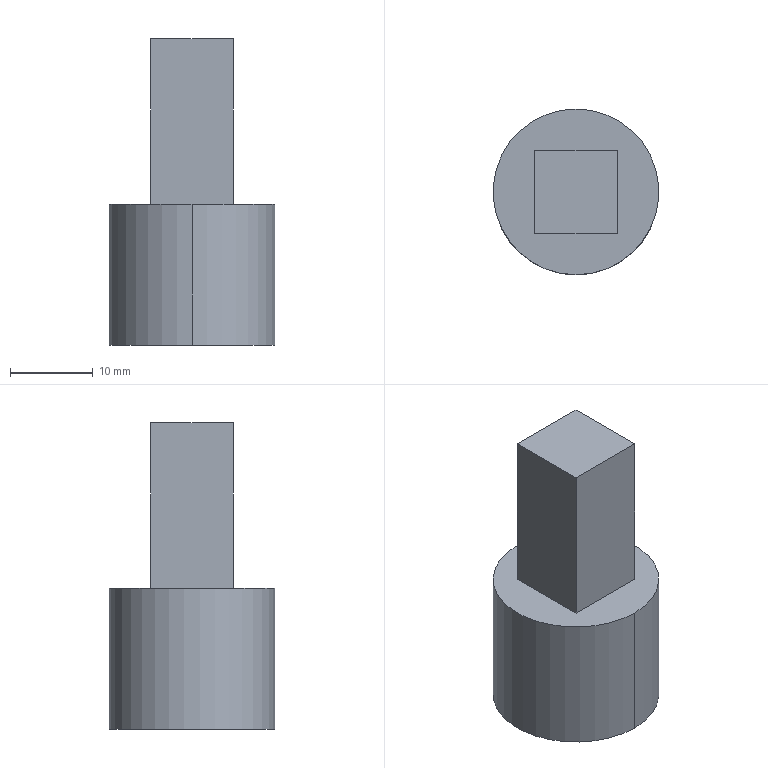Component | SolidWorks | MotorDriveShaft-1 | 1 solid | 12 faces | box 20 x 20 x 37 mm | volume 5032 mm3 | plane 8 | cylinder 4 | commonest cylinder face diameters 14 x2 20 x2
build123d program:
from build123d import *

# Parameters (mm, degrees)
SKETCH1_W           = 10
SKETCH1_H           = 10
BOSS_EXTRUDE1_DEPTH = 20
SKETCH2_R           = 10
BOSS_EXTRUDE2_DEPTH = 2
SKETCH3_R           = 10
SKETCH3_R_2         = 7
BOSS_EXTRUDE3_DEPTH = 15


with BuildPart() as part:
    # Sketch1 → Boss-Extrude1 (new body)
    with BuildSketch(Plane.XY):
        Rectangle(SKETCH1_W, SKETCH1_H)
    extrude(amount=BOSS_EXTRUDE1_DEPTH)

    # Sketch2 → Boss-Extrude2 (add)
    with BuildSketch(Plane.XY.offset(20)):
        Circle(SKETCH2_R)
    extrude(amount=BOSS_EXTRUDE2_DEPTH)

    # Sketch3 → Boss-Extrude3 (add)
    with BuildSketch(Plane.XY.offset(22)):
        Circle(SKETCH3_R)
        Circle(SKETCH3_R_2, mode=Mode.SUBTRACT)
    extrude(amount=BOSS_EXTRUDE3_DEPTH)


solid = part.part

# Placed as in the assembly
solid = solid.moved(Location((-65.193, -32.853, 1589.064), (180, 0, 0)))
STEP:
#1=CARTESIAN_POINT('',(-2.567,-1.018,61.105));
#2=VERTEX_POINT('',#1);
#3=CARTESIAN_POINT('',(-2.567,-1.569,61.105));
#4=VERTEX_POINT('',#3);
#5=CARTESIAN_POINT('',(-2.567,-1.293,61.105));
#6=DIRECTION('',(-0.,-0.,-1.));
#7=DIRECTION('',(0.,-1.,0.));
#8=AXIS2_PLACEMENT_3D('',#5,#6,#7);
#9=CIRCLE('',#8,0.2756);
#10=EDGE_CURVE('',#2,#4,#9,.T.);
#11=ORIENTED_EDGE('',*,*,#10,.T.);
#12=CARTESIAN_POINT('',(-2.567,-1.569,61.695));
#13=VERTEX_POINT('',#12);
#14=CARTESIAN_POINT('',(-2.567,-1.569,61.105));
#15=DIRECTION('',(0.,0.,1.));
#16=VECTOR('',#15,39.37);
#17=LINE('',#14,#16);
#18=EDGE_CURVE('',#4,#13,#17,.T.);
#19=ORIENTED_EDGE('',*,*,#18,.T.);
#20=CARTESIAN_POINT('',(-2.567,-1.018,61.695));
#21=VERTEX_POINT('',#20);
#22=CARTESIAN_POINT('',(-2.567,-1.293,61.695));
#23=DIRECTION('',(0.,0.,1.));
#24=DIRECTION('',(0.,-1.,0.));
#25=AXIS2_PLACEMENT_3D('',#22,#23,#24);
#26=CIRCLE('',#25,0.2756);
#27=EDGE_CURVE('',#13,#21,#26,.T.);
#28=ORIENTED_EDGE('',*,*,#27,.T.);
#29=CARTESIAN_POINT('',(-2.567,-1.018,61.105));
#30=DIRECTION('',(0.,0.,1.));
#31=VECTOR('',#30,39.37);
#32=LINE('',#29,#31);
#33=EDGE_CURVE('',#2,#21,#32,.T.);
#34=ORIENTED_EDGE('',*,*,#33,.F.);
#35=EDGE_LOOP('',(#11,#19,#28,#34));
#36=FACE_OUTER_BOUND('',#35,.T.);
#37=CARTESIAN_POINT('',(-2.567,-1.293,61.105));
#38=DIRECTION('',(0.,0.,1.));
#39=DIRECTION('',(0.,1.,0.));
#40=AXIS2_PLACEMENT_3D('',#37,#38,#39);
#41=CYLINDRICAL_SURFACE('',#40,0.2756);
#42=ADVANCED_FACE('',(#36),#41,.F.);
#43=CARTESIAN_POINT('',(-2.567,-1.687,61.105));
#44=VERTEX_POINT('',#43);
#45=CARTESIAN_POINT('',(-2.567,-0.8997,61.105));
#46=VERTEX_POINT('',#45);
#47=CARTESIAN_POINT('',(-2.567,-1.293,61.105));
#48=DIRECTION('',(-0.,-0.,-1.));
#49=DIRECTION('',(0.,-1.,0.));
#50=AXIS2_PLACEMENT_3D('',#47,#48,#49);
#51=CIRCLE('',#50,0.3937);
#52=EDGE_CURVE('',#44,#46,#51,.T.);
#53=ORIENTED_EDGE('',*,*,#52,.F.);
#54=CARTESIAN_POINT('',(-2.567,-1.687,61.774));
#55=VERTEX_POINT('',#54);
#56=CARTESIAN_POINT('',(-2.567,-1.687,61.695));
#57=DIRECTION('',(0.,0.,1.));
#58=VECTOR('',#57,39.37);
#59=LINE('',#56,#58);
#60=EDGE_CURVE('',#44,#55,#59,.T.);
#61=ORIENTED_EDGE('',*,*,#60,.T.);
#62=CARTESIAN_POINT('',(-2.567,-0.8997,61.774));
#63=VERTEX_POINT('',#62);
#64=CARTESIAN_POINT('',(-2.567,-1.293,61.774));
#65=DIRECTION('',(-0.,-0.,-1.));
#66=DIRECTION('',(0.,-1.,0.));
#67=AXIS2_PLACEMENT_3D('',#64,#65,#66);
#68=CIRCLE('',#67,0.3937);
#69=EDGE_CURVE('',#55,#63,#68,.T.);
#70=ORIENTED_EDGE('',*,*,#69,.T.);
#71=CARTESIAN_POINT('',(-2.567,-0.8997,61.695));
#72=DIRECTION('',(0.,0.,1.));
#73=VECTOR('',#72,39.37);
#74=LINE('',#71,#73);
#75=EDGE_CURVE('',#46,#63,#74,.T.);
#76=ORIENTED_EDGE('',*,*,#75,.F.);
#77=EDGE_LOOP('',(#53,#61,#70,#76));
#78=FACE_OUTER_BOUND('',#77,.T.);
#79=CARTESIAN_POINT('',(-2.567,-1.293,61.695));
#80=DIRECTION('',(0.,0.,1.));
#81=DIRECTION('',(0.,1.,0.));
#82=AXIS2_PLACEMENT_3D('',#79,#80,#81);
#83=CYLINDRICAL_SURFACE('',#82,0.3937);
#84=ADVANCED_FACE('',(#78),#83,.T.);
#85=CARTESIAN_POINT('',(-2.37,-1.49,62.562));
#86=VERTEX_POINT('',#85);
#87=CARTESIAN_POINT('',(-2.764,-1.49,62.562));
#88=VERTEX_POINT('',#87);
#89=CARTESIAN_POINT('',(-2.764,-1.49,62.562));
#90=DIRECTION('',(-1.,0.,0.));
#91=VECTOR('',#90,39.37);
#92=LINE('',#89,#91);
#93=EDGE_CURVE('',#86,#88,#92,.T.);
#94=ORIENTED_EDGE('',*,*,#93,.T.);
#95=CARTESIAN_POINT('',(-2.764,-1.49,61.774));
#96=VERTEX_POINT('',#95);
#97=CARTESIAN_POINT('',(-2.764,-1.49,61.774));
#98=DIRECTION('',(0.,0.,1.));
#99=VECTOR('',#98,39.37);
#100=LINE('',#97,#99);
#101=EDGE_CURVE('',#96,#88,#100,.T.);
#102=ORIENTED_EDGE('',*,*,#101,.F.);
#103=CARTESIAN_POINT('',(-2.37,-1.49,61.774));
#104=VERTEX_POINT('',#103);
#105=CARTESIAN_POINT('',(-2.764,-1.49,61.774));
#106=DIRECTION('',(-1.,0.,0.));
#107=VECTOR('',#106,39.37);
#108=LINE('',#105,#107);
#109=EDGE_CURVE('',#104,#96,#108,.T.);
#110=ORIENTED_EDGE('',*,*,#109,.F.);
#111=CARTESIAN_POINT('',(-2.37,-1.49,61.774));
#112=DIRECTION('',(0.,0.,1.));
#113=VECTOR('',#112,39.37);
#114=LINE('',#111,#113);
#115=EDGE_CURVE('',#104,#86,#114,.T.);
#116=ORIENTED_EDGE('',*,*,#115,.T.);
#117=EDGE_LOOP('',(#94,#102,#110,#116));
#118=FACE_OUTER_BOUND('',#117,.T.);
#119=CARTESIAN_POINT('',(-2.764,-1.49,61.774));
#120=DIRECTION('',(0.,1.,-0.));
#121=DIRECTION('',(1.,-0.,-0.));
#122=AXIS2_PLACEMENT_3D('',#119,#120,#121);
#123=PLANE('',#122);
#124=ADVANCED_FACE('',(#118),#123,.F.);
#125=CARTESIAN_POINT('',(-2.764,-1.097,62.562));
#126=VERTEX_POINT('',#125);
#127=CARTESIAN_POINT('',(-2.764,-1.097,62.562));
#128=DIRECTION('',(-0.,1.,-0.));
#129=VECTOR('',#128,39.37);
#130=LINE('',#127,#129);
#131=EDGE_CURVE('',#88,#126,#130,.T.);
#132=ORIENTED_EDGE('',*,*,#131,.T.);
#133=CARTESIAN_POINT('',(-2.764,-1.097,61.774));
#134=VERTEX_POINT('',#133);
#135=CARTESIAN_POINT('',(-2.764,-1.097,61.774));
#136=DIRECTION('',(0.,0.,1.));
#137=VECTOR('',#136,39.37);
#138=LINE('',#135,#137);
#139=EDGE_CURVE('',#134,#126,#138,.T.);
#140=ORIENTED_EDGE('',*,*,#139,.F.);
#141=CARTESIAN_POINT('',(-2.764,-1.097,61.774));
#142=DIRECTION('',(-0.,1.,-0.));
#143=VECTOR('',#142,39.37);
#144=LINE('',#141,#143);
#145=EDGE_CURVE('',#96,#134,#144,.T.);
#146=ORIENTED_EDGE('',*,*,#145,.F.);
#147=ORIENTED_EDGE('',*,*,#101,.T.);
#148=EDGE_LOOP('',(#132,#140,#146,#147));
#149=FACE_OUTER_BOUND('',#148,.T.);
#150=CARTESIAN_POINT('',(-2.764,-1.097,61.774));
#151=DIRECTION('',(1.,0.,-0.));
#152=DIRECTION('',(0.,-1.,0.));
#153=AXIS2_PLACEMENT_3D('',#150,#151,#152);
#154=PLANE('',#153);
#155=ADVANCED_FACE('',(#149),#154,.F.);
#156=CARTESIAN_POINT('',(-2.37,-1.097,62.562));
#157=VERTEX_POINT('',#156);
#158=CARTESIAN_POINT('',(-2.764,-1.097,62.562));
#159=DIRECTION('',(1.,-0.,-0.));
#160=VECTOR('',#159,39.37);
#161=LINE('',#158,#160);
#162=EDGE_CURVE('',#126,#157,#161,.T.);
#163=ORIENTED_EDGE('',*,*,#162,.T.);
#164=CARTESIAN_POINT('',(-2.37,-1.097,61.774));
#165=VERTEX_POINT('',#164);
#166=CARTESIAN_POINT('',(-2.37,-1.097,61.774));
#167=DIRECTION('',(0.,0.,1.));
#168=VECTOR('',#167,39.37);
#169=LINE('',#166,#168);
#170=EDGE_CURVE('',#165,#157,#169,.T.);
#171=ORIENTED_EDGE('',*,*,#170,.F.);
#172=CARTESIAN_POINT('',(-2.764,-1.097,61.774));
#173=DIRECTION('',(1.,-0.,-0.));
#174=VECTOR('',#173,39.37);
#175=LINE('',#172,#174);
#176=EDGE_CURVE('',#134,#165,#175,.T.);
#177=ORIENTED_EDGE('',*,*,#176,.F.);
#178=ORIENTED_EDGE('',*,*,#139,.T.);
#179=EDGE_LOOP('',(#163,#171,#177,#178));
#180=FACE_OUTER_BOUND('',#179,.T.);
#181=CARTESIAN_POINT('',(-2.764,-1.097,61.774));
#182=DIRECTION('',(-0.,-1.,0.));
#183=DIRECTION('',(-1.,0.,0.));
#184=AXIS2_PLACEMENT_3D('',#181,#182,#183);
#185=PLANE('',#184);
#186=ADVANCED_FACE('',(#180),#185,.F.);
#187=CARTESIAN_POINT('',(-2.37,-1.097,62.562));
#188=DIRECTION('',(-0.,-1.,0.));
#189=VECTOR('',#188,39.37);
#190=LINE('',#187,#189);
#191=EDGE_CURVE('',#157,#86,#190,.T.);
#192=ORIENTED_EDGE('',*,*,#191,.T.);
#193=ORIENTED_EDGE('',*,*,#115,.F.);
#194=CARTESIAN_POINT('',(-2.37,-1.097,61.774));
#195=DIRECTION('',(-0.,-1.,0.));
#196=VECTOR('',#195,39.37);
#197=LINE('',#194,#196);
#198=EDGE_CURVE('',#165,#104,#197,.T.);
#199=ORIENTED_EDGE('',*,*,#198,.F.);
#200=ORIENTED_EDGE('',*,*,#170,.T.);
#201=EDGE_LOOP('',(#192,#193,#199,#200));
#202=FACE_OUTER_BOUND('',#201,.T.);
#203=CARTESIAN_POINT('',(-2.37,-1.097,61.774));
#204=DIRECTION('',(-1.,0.,0.));
#205=DIRECTION('',(-0.,-0.,-1.));
#206=AXIS2_PLACEMENT_3D('',#203,#204,#205);
#207=PLANE('',#206);
#208=ADVANCED_FACE('',(#202),#207,.F.);
#209=ORIENTED_EDGE('',*,*,#93,.F.);
#210=ORIENTED_EDGE('',*,*,#191,.F.);
#211=ORIENTED_EDGE('',*,*,#162,.F.);
#212=ORIENTED_EDGE('',*,*,#131,.F.);
#213=EDGE_LOOP('',(#209,#210,#211,#212));
#214=FACE_OUTER_BOUND('',#213,.T.);
#215=CARTESIAN_POINT('',(-2.567,-1.293,62.562));
#216=DIRECTION('',(-0.,-0.,-1.));
#217=DIRECTION('',(-0.,-1.,0.));
#218=AXIS2_PLACEMENT_3D('',#215,#216,#217);
#219=PLANE('',#218);
#220=ADVANCED_FACE('',(#214),#219,.F.);
#221=CARTESIAN_POINT('',(-2.567,-1.293,61.774));
#222=DIRECTION('',(-0.,-0.,-1.));
#223=DIRECTION('',(0.,-1.,0.));
#224=AXIS2_PLACEMENT_3D('',#221,#222,#223);
#225=CIRCLE('',#224,0.3937);
#226=EDGE_CURVE('',#63,#55,#225,.T.);
#227=ORIENTED_EDGE('',*,*,#226,.F.);
#228=ORIENTED_EDGE('',*,*,#69,.F.);
#229=EDGE_LOOP('',(#227,#228));
#230=FACE_OUTER_BOUND('',#229,.T.);
#231=ORIENTED_EDGE('',*,*,#198,.T.);
#232=ORIENTED_EDGE('',*,*,#109,.T.);
#233=ORIENTED_EDGE('',*,*,#145,.T.);
#234=ORIENTED_EDGE('',*,*,#176,.T.);
#235=EDGE_LOOP('',(#231,#232,#233,#234));
#236=FACE_BOUND('',#235,.T.);
#237=CARTESIAN_POINT('',(-2.567,-1.293,61.774));
#238=DIRECTION('',(-0.,-0.,-1.));
#239=DIRECTION('',(-0.,-1.,0.));
#240=AXIS2_PLACEMENT_3D('',#237,#238,#239);
#241=PLANE('',#240);
#242=ADVANCED_FACE('',(#230,#236),#241,.F.);
#243=ORIENTED_EDGE('',*,*,#60,.F.);
#244=CARTESIAN_POINT('',(-2.567,-1.293,61.105));
#245=DIRECTION('',(-0.,-0.,-1.));
#246=DIRECTION('',(0.,-1.,0.));
#247=AXIS2_PLACEMENT_3D('',#244,#245,#246);
#248=CIRCLE('',#247,0.3937);
#249=EDGE_CURVE('',#46,#44,#248,.T.);
#250=ORIENTED_EDGE('',*,*,#249,.F.);
#251=ORIENTED_EDGE('',*,*,#75,.T.);
#252=ORIENTED_EDGE('',*,*,#226,.T.);
#253=EDGE_LOOP('',(#243,#250,#251,#252));
#254=FACE_OUTER_BOUND('',#253,.T.);
#255=CARTESIAN_POINT('',(-2.567,-1.293,61.695));
#256=DIRECTION('',(0.,0.,1.));
#257=DIRECTION('',(0.,1.,0.));
#258=AXIS2_PLACEMENT_3D('',#255,#256,#257);
#259=CYLINDRICAL_SURFACE('',#258,0.3937);
#260=ADVANCED_FACE('',(#254),#259,.T.);
#261=ORIENTED_EDGE('',*,*,#249,.T.);
#262=ORIENTED_EDGE('',*,*,#52,.T.);
#263=EDGE_LOOP('',(#261,#262));
#264=FACE_OUTER_BOUND('',#263,.T.);
#265=ORIENTED_EDGE('',*,*,#10,.F.);
#266=CARTESIAN_POINT('',(-2.567,-1.293,61.105));
#267=DIRECTION('',(-0.,-0.,-1.));
#268=DIRECTION('',(0.,-1.,0.));
#269=AXIS2_PLACEMENT_3D('',#266,#267,#268);
#270=CIRCLE('',#269,0.2756);
#271=EDGE_CURVE('',#4,#2,#270,.T.);
#272=ORIENTED_EDGE('',*,*,#271,.F.);
#273=EDGE_LOOP('',(#265,#272));
#274=FACE_BOUND('',#273,.T.);
#275=CARTESIAN_POINT('',(-2.567,-1.293,61.105));
#276=DIRECTION('',(-0.,-0.,-1.));
#277=DIRECTION('',(-0.,-1.,0.));
#278=AXIS2_PLACEMENT_3D('',#275,#276,#277);
#279=PLANE('',#278);
#280=ADVANCED_FACE('',(#264,#274),#279,.T.);
#281=ORIENTED_EDGE('',*,*,#18,.F.);
#282=ORIENTED_EDGE('',*,*,#271,.T.);
#283=ORIENTED_EDGE('',*,*,#33,.T.);
#284=CARTESIAN_POINT('',(-2.567,-1.293,61.695));
#285=DIRECTION('',(0.,0.,1.));
#286=DIRECTION('',(0.,-1.,0.));
#287=AXIS2_PLACEMENT_3D('',#284,#285,#286);
#288=CIRCLE('',#287,0.2756);
#289=EDGE_CURVE('',#21,#13,#288,.T.);
#290=ORIENTED_EDGE('',*,*,#289,.T.);
#291=EDGE_LOOP('',(#281,#282,#283,#290));
#292=FACE_OUTER_BOUND('',#291,.T.);
#293=CARTESIAN_POINT('',(-2.567,-1.293,61.105));
#294=DIRECTION('',(0.,0.,1.));
#295=DIRECTION('',(0.,1.,0.));
#296=AXIS2_PLACEMENT_3D('',#293,#294,#295);
#297=CYLINDRICAL_SURFACE('',#296,0.2756);
#298=ADVANCED_FACE('',(#292),#297,.F.);
#299=ORIENTED_EDGE('',*,*,#289,.F.);
#300=ORIENTED_EDGE('',*,*,#27,.F.);
#301=EDGE_LOOP('',(#299,#300));
#302=FACE_OUTER_BOUND('',#301,.T.);
#303=CARTESIAN_POINT('',(-2.567,-1.293,61.695));
#304=DIRECTION('',(-0.,-0.,-1.));
#305=DIRECTION('',(-0.,-1.,0.));
#306=AXIS2_PLACEMENT_3D('',#303,#304,#305);
#307=PLANE('',#306);
#308=ADVANCED_FACE('',(#302),#307,.T.);
#309=CLOSED_SHELL('',(#42,#84,#124,#155,#186,#208,#220,#242,#260,#280,#298,#308));
#310=MANIFOLD_SOLID_BREP('',#309);
#311=CARTESIAN_POINT('',(0.,0.,0.));
#312=DIRECTION('',(0.,0.,1.));
#313=DIRECTION('',(1.,0.,0.));
#314=AXIS2_PLACEMENT_3D('',#311,#312,#313);
#315=(LENGTH_UNIT()NAMED_UNIT(*)SI_UNIT($,.METRE.));
#316=LENGTH_MEASURE_WITH_UNIT(LENGTH_MEASURE(0.0254),#315);
#317=DIMENSIONAL_EXPONENTS(1.,0.,0.,0.,0.,0.,0.);
#318=(CONVERSION_BASED_UNIT('',#316)LENGTH_UNIT()NAMED_UNIT(#317));
#319=UNCERTAINTY_MEASURE_WITH_UNIT(LENGTH_MEASURE(0.00001),#318,'','');
#320=(NAMED_UNIT(*)PLANE_ANGLE_UNIT()SI_UNIT($,.RADIAN.));
#321=(NAMED_UNIT(*)SI_UNIT($,.STERADIAN.)SOLID_ANGLE_UNIT());
#322=(GEOMETRIC_REPRESENTATION_CONTEXT(3)GLOBAL_UNCERTAINTY_ASSIGNED_CONTEXT((#319))GLOBAL_UNIT_ASSIGNED_CONTEXT((#318,#320,#321))REPRESENTATION_CONTEXT('',''));
#323=ADVANCED_BREP_SHAPE_REPRESENTATION('',(#310,#314),#322);
#324=COLOUR_RGB('',0.7922,0.8196,0.9333);
#325=FILL_AREA_STYLE_COLOUR('',#324);
#326=FILL_AREA_STYLE('',(#325));
#327=SURFACE_STYLE_FILL_AREA(#326);
#328=SURFACE_SIDE_STYLE('',(#327));
#329=SURFACE_STYLE_USAGE(.BOTH.,#328);
#330=PRESENTATION_STYLE_ASSIGNMENT((#329));
#331=STYLED_ITEM('',(#330),#310);
#332=PRESENTATION_LAYER_ASSIGNMENT('','',(#331));
#333=(LENGTH_UNIT()NAMED_UNIT(*)SI_UNIT($,.METRE.));
#334=LENGTH_MEASURE_WITH_UNIT(LENGTH_MEASURE(0.0254),#333);
#335=DIMENSIONAL_EXPONENTS(1.,0.,0.,0.,0.,0.,0.);
#336=(CONVERSION_BASED_UNIT('',#334)LENGTH_UNIT()NAMED_UNIT(#335));
#337=UNCERTAINTY_MEASURE_WITH_UNIT(LENGTH_MEASURE(0.00001),#336,'','');
#338=(NAMED_UNIT(*)PLANE_ANGLE_UNIT()SI_UNIT($,.RADIAN.));
#339=(NAMED_UNIT(*)SI_UNIT($,.STERADIAN.)SOLID_ANGLE_UNIT());
#340=(GEOMETRIC_REPRESENTATION_CONTEXT(3)GLOBAL_UNCERTAINTY_ASSIGNED_CONTEXT((#337))GLOBAL_UNIT_ASSIGNED_CONTEXT((#336,#338,#339))REPRESENTATION_CONTEXT('',''));
#341=MECHANICAL_DESIGN_GEOMETRIC_PRESENTATION_REPRESENTATION('',(#331),#340);